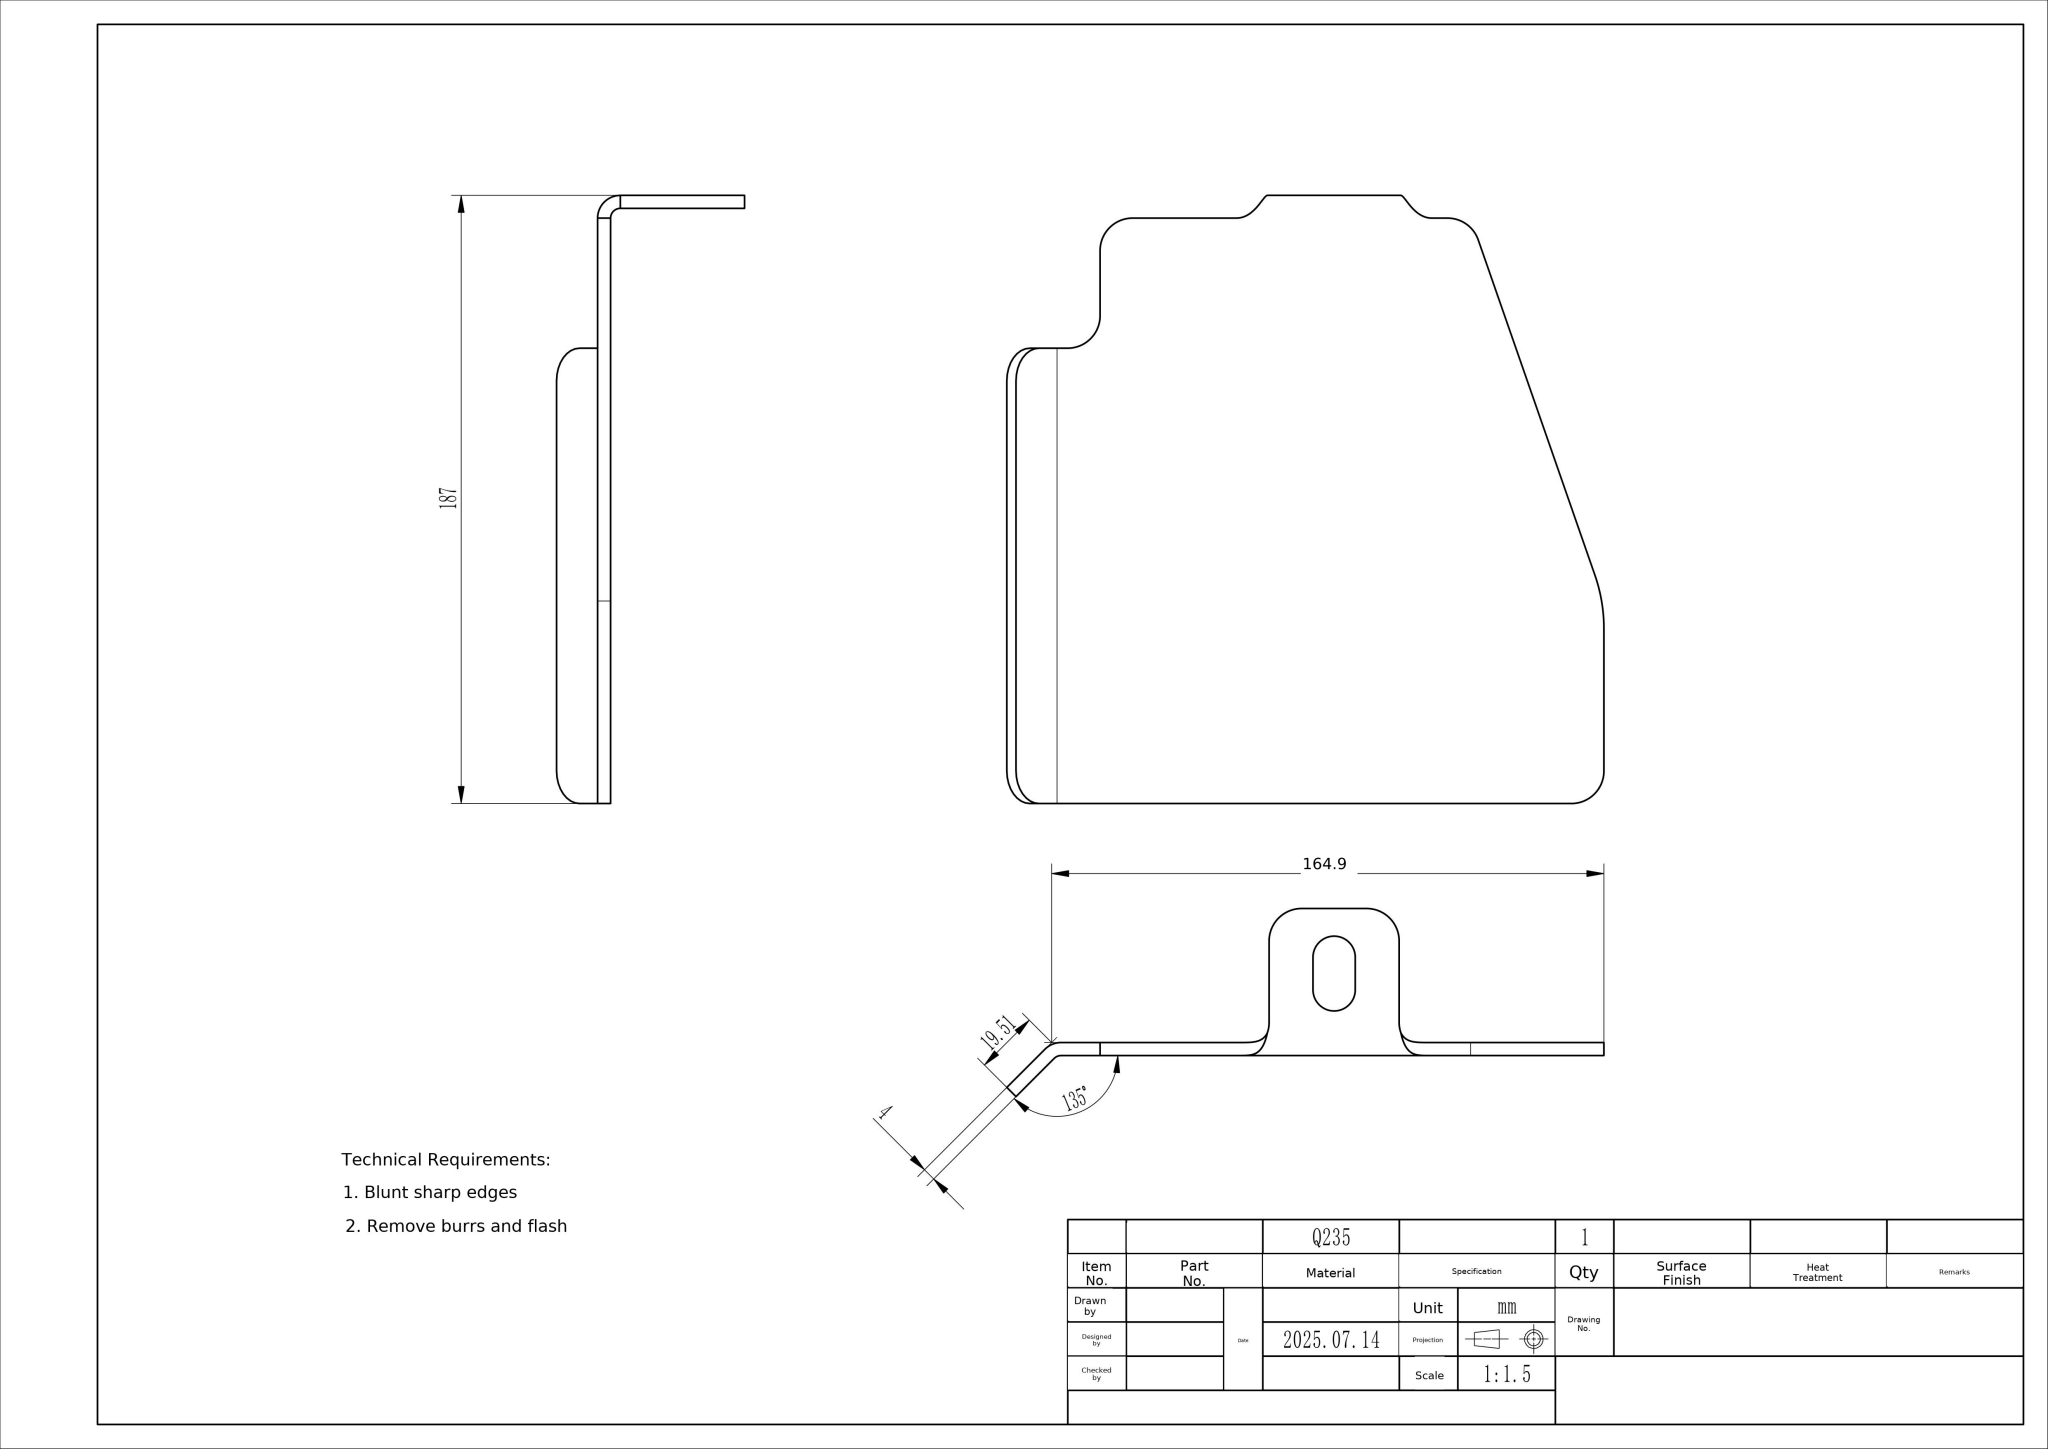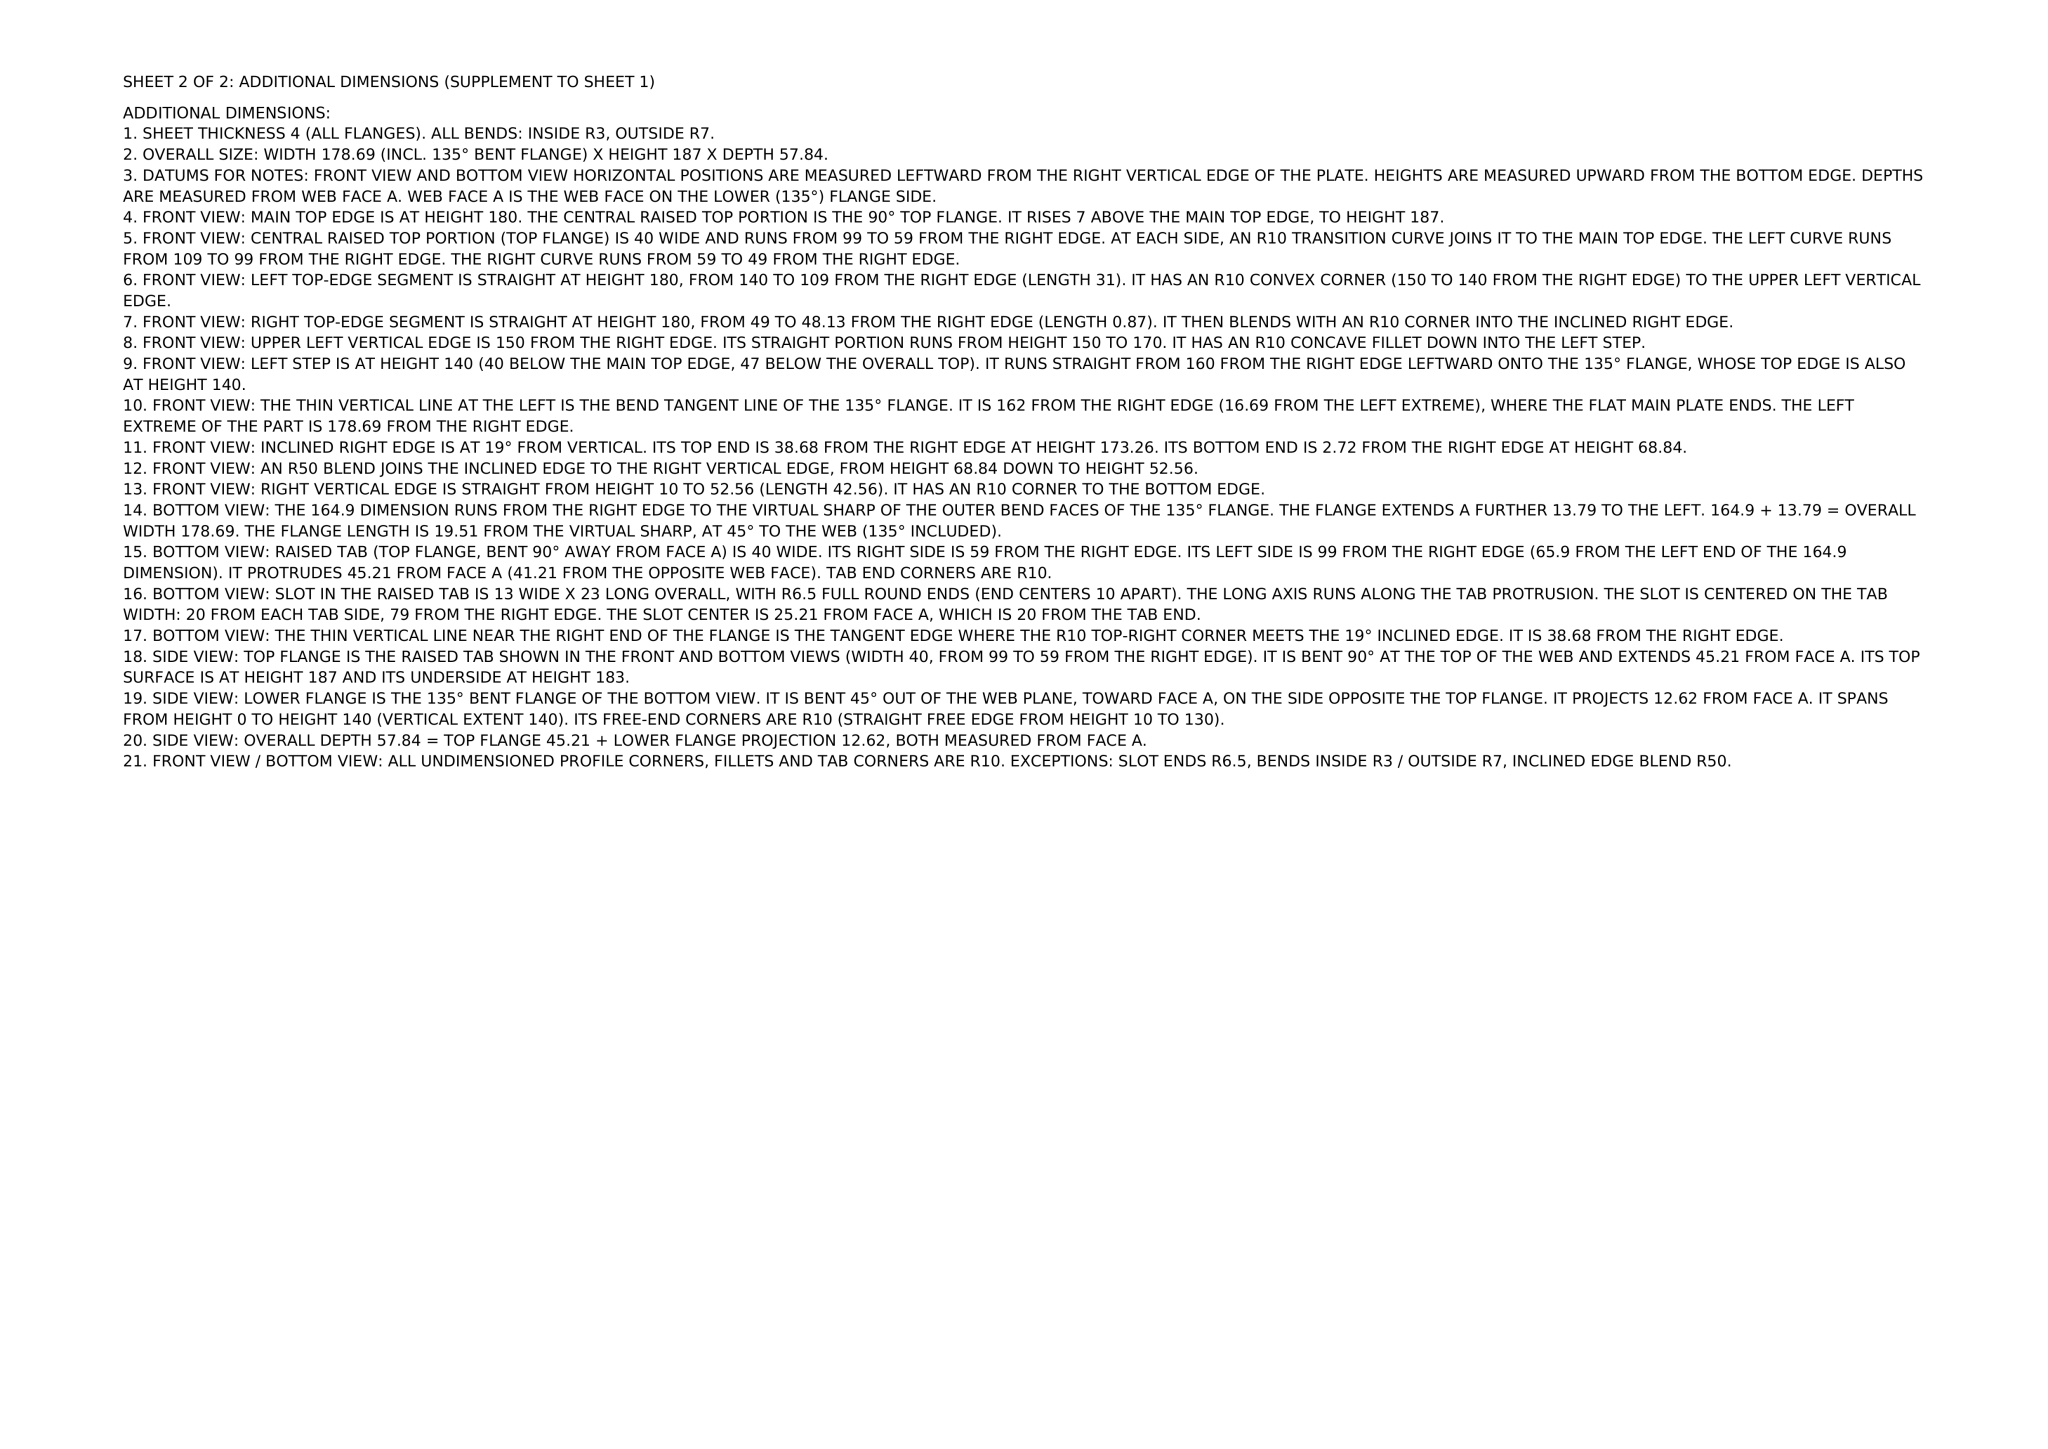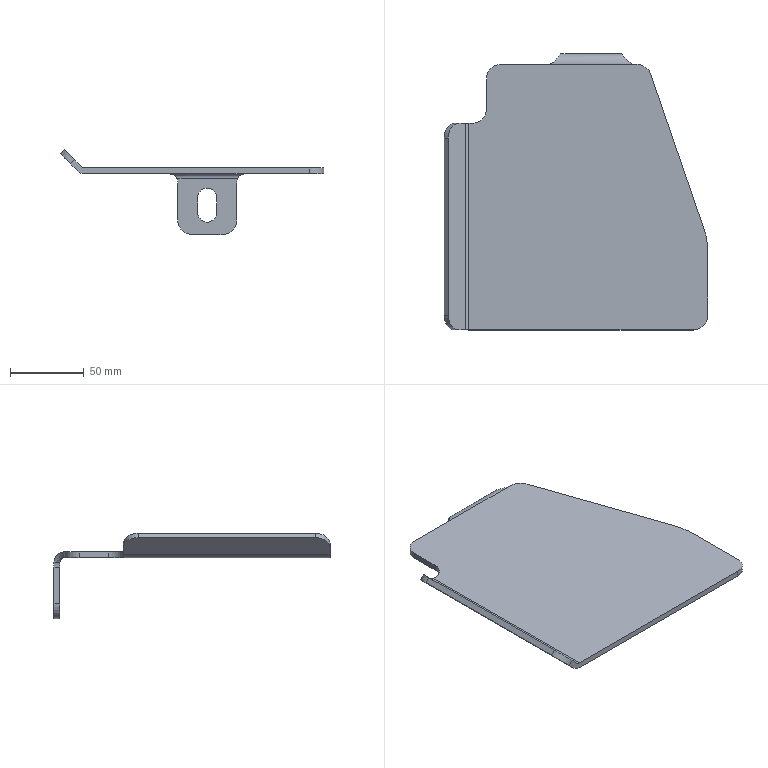Part | NX | mm | 1 solid | 38 faces | box 178.69 x 187 x 57.84 mm | volume 122491 mm3 | plane 19 | cylinder 17 | spline 2 | commonest cylinder face diameters 20 x10 13 x2 14 x2 6 x2 100 x1